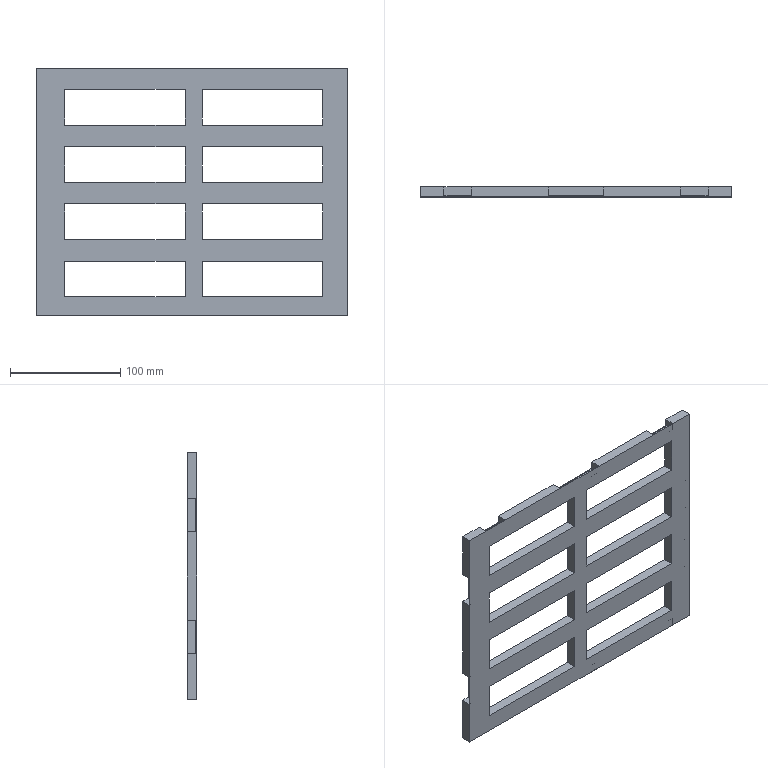Component | SolidWorks | 2011FeederTray-1 | 1 solid | 311 faces | box 282 x 9 x 224 mm | volume 294343 mm3 | plane 214 | spline 97
build123d program:
from build123d import *

# Parameters (mm, degrees)
SKETCH1_W            = 282
SKETCH1_H            = 224
BOSS_EXTRUDE1_DEPTH  = 9
SKETCH2_W            = 25
SKETCH2_H            = 7
SKETCH2_W_2          = 50
CUT_EXTRUDE1_DEPTH   = 8
SKETCH3_W            = 7
SKETCH3_H            = 30
CUT_EXTRUDE2_DEPTH   = 8
SKETCH4_W            = 7
SKETCH4_H            = 30
CUT_EXTRUDE3_DEPTH   = 8
SKETCH5_W            = 109.5
SKETCH5_H            = 32.5
CUT_EXTRUDE4_DEPTH   = 9
LPATTERN1_COUNT      = 4
LPATTERN1_PITCH      = 52
LPATTERN1_COUNT_DIR2 = 2
LPATTERN1_PITCH_DIR2 = 125
CUT_EXTRUDE5_DEPTH   = 2


with BuildPart() as part:
    # Sketch1 → Boss-Extrude1 (new body)
    with BuildSketch(Plane.XY):
        with Locations((141, 112)):
            Rectangle(SKETCH1_W, SKETCH1_H)
    extrude(amount=BOSS_EXTRUDE1_DEPTH)

    # Sketch2 → Cut-Extrude1 (cut)
    with BuildSketch(Plane(origin=(0, 0, 0), x_dir=(-1, 0, 0), z_dir=(0, 0, -1))):
        with Locations((-248.5, 3.5)):
            Rectangle(SKETCH2_W, SKETCH2_H)
        with Locations((-141, 3.5)):
            Rectangle(SKETCH2_W_2, SKETCH2_H)
        with Locations((-33.5, 3.5)):
            Rectangle(SKETCH2_W, SKETCH2_H)
    cut_extrude1 = extrude(amount=-CUT_EXTRUDE1_DEPTH, mode=Mode.SUBTRACT)

    # Mirror1: Cut-Extrude1 across plane
    add(cut_extrude1.mirror(Plane.ZX.offset(112)), mode=Mode.SUBTRACT)

    # Sketch3 → Cut-Extrude2 (cut)
    with BuildSketch(Plane(origin=(0, 0, 0), x_dir=(-1, 0, 0), z_dir=(0, 0, -1))):
        with Locations((-278.5, 167)):
            Rectangle(SKETCH3_W, SKETCH3_H)
        with Locations((-278.5, 57)):
            Rectangle(SKETCH3_W, SKETCH3_H)
    extrude(amount=-CUT_EXTRUDE2_DEPTH, mode=Mode.SUBTRACT)

    # Sketch4 → Cut-Extrude3 (cut)
    with BuildSketch(Plane(origin=(0, 0, 0), x_dir=(-1, 0, 0), z_dir=(0, 0, -1))):
        with Locations((-3.5, 152)):
            Rectangle(SKETCH4_W, SKETCH4_H)
        with Locations((-3.5, 87)):
            Rectangle(SKETCH4_W, SKETCH4_H)
    extrude(amount=-CUT_EXTRUDE3_DEPTH, mode=Mode.SUBTRACT)

    # Sketch5 → Cut-Extrude4 (cut)
    with BuildSketch(Plane(origin=(0, 0, 0), x_dir=(-1, 0, 0), z_dir=(0, 0, -1))):
        with Locations((-77, 191)):
            Rectangle(SKETCH5_W, SKETCH5_H)
    cut_extrude4 = extrude(amount=-CUT_EXTRUDE4_DEPTH, mode=Mode.SUBTRACT)

    # LPattern1: Cut-Extrude4 4 × 2
    with Locations(*[(j * LPATTERN1_PITCH_DIR2, -i * LPATTERN1_PITCH, 0) for i in range(LPATTERN1_COUNT) for j in range(LPATTERN1_COUNT_DIR2) if (i, j) != (0, 0)]):
        add(cut_extrude4, mode=Mode.SUBTRACT)

    # Sketch7 → Cut-Extrude5 (cut)
    # profile 1 of 6: a face of its own
    with BuildSketch(Plane(origin=(0, 0, 0), x_dir=(-1, 0, 0), z_dir=(0, 0, -1))):
        with BuildLine():
            add(Edge.make_bspline(
                [(-22.181, 112.918), (-22.127, 113.019), (-22.02, 113.218), (-21.9, 113.472), (-21.811, 113.669), (-21.753, 113.809), (-21.7, 113.94), (-21.659, 114.046), (-21.63, 114.13), (-21.607, 114.198), (-21.584, 114.273), (-21.56, 114.353), (-21.534, 114.439), (-21.509, 114.531), (-21.482, 114.629), (-21.465, 114.696), (-21.456, 114.731)],
                knots=[0, 0, 0, 0, 2.447, 4.852, 6.014, 7.097, 8.109, 9.044, 9.513, 10.031, 10.584, 11.185, 11.824, 12.505, 13.234, 14, 14, 14, 14], degree=3))
            add(Edge.make_bspline(
                [(-21.456, 114.731), (-21.484, 114.723), (-21.536, 114.708), (-21.611, 114.687), (-21.678, 114.666), (-21.738, 114.649), (-21.789, 114.631), (-21.833, 114.617), (-21.869, 114.603), (-21.89, 114.594), (-21.899, 114.59)],
                knots=[0, 0, 0, 0, 1.478, 2.813, 4.018, 5.09, 6.022, 6.809, 7.471, 8, 8, 8, 8], degree=3))
            Line((-21.899, 114.59), (-22.02, 114.716))
            add(Edge.make_bspline(
                [(-22.02, 114.716), (-22.028, 114.724), (-22.039, 114.737), (-22.055, 114.755), (-22.051, 114.772), (-22.044, 114.778), (-22.04, 114.781)],
                knots=[0, 0, 0, 0, 1.714, 2.651, 3.248, 4, 4, 4, 4], degree=3))
            add(Edge.make_bspline(
                [(-22.04, 114.781), (-22.038, 114.783), (-22.028, 114.787), (-22.014, 114.783), (-21.996, 114.783), (-21.977, 114.786), (-21.951, 114.791), (-21.917, 114.796), (-21.875, 114.803), (-21.826, 114.813), (-21.769, 114.824), (-21.729, 114.832), (-21.708, 114.837)],
                knots=[0, 0, 0, 0, 0.2376, 0.8998, 1.231, 1.808, 2.592, 3.618, 4.873, 6.357, 8.066, 10, 10, 10, 10], degree=3))
            Line((-21.708, 114.837), (-21.4, 114.897))
            Line((-21.4, 114.897), (-21.396, 115.541))
            Line((-21.396, 115.541), (-21.396, 115.657))
            add(Edge.make_bspline(
                [(-21.396, 115.657), (-21.396, 115.673), (-21.396, 115.702), (-21.396, 115.738), (-21.396, 115.762), (-21.396, 115.774), (-21.396, 115.778)],
                knots=[0, 0, 0, 0, 1.63, 2.84, 3.63, 4, 4, 4, 4], degree=3))
            add(Edge.make_bspline(
                [(-21.396, 115.778), (-21.396, 115.785), (-21.396, 115.805), (-21.398, 115.838), (-21.399, 115.883), (-21.402, 115.953), (-21.406, 116.039), (-21.41, 116.122), (-21.42, 116.187), (-21.431, 116.247), (-21.45, 116.32), (-21.464, 116.373), (-21.471, 116.402)],
                knots=[0, 0, 0, 0, 0.3663, 0.9103, 1.608, 2.483, 4.245, 5.679, 6.431, 7.392, 8.584, 10, 10, 10, 10], degree=3))
            Line((-21.471, 116.402), (-21.436, 116.442))
            Line((-21.436, 116.442), (-21.169, 116.11))
            add(Edge.make_bspline(
                [(-21.169, 116.11), (-21.179, 116.086), (-21.197, 116.038), (-21.224, 115.966), (-21.243, 115.887), (-21.253, 115.795), (-21.258, 115.687), (-21.263, 115.565), (-21.264, 115.439), (-21.264, 115.355), (-21.265, 115.315)],
                knots=[0, 0, 0, 0, 0.7826, 1.518, 2.286, 3.193, 4.257, 5.505, 6.797, 8, 8, 8, 8], degree=3))
            Line((-21.265, 115.315), (-21.27, 114.932))
            Line((-21.27, 114.932), (-21.159, 114.963))
            add(Edge.make_bspline(
                [(-21.159, 114.963), (-21.131, 114.97), (-21.08, 114.984), (-21.012, 115.011), (-20.956, 115.038), (-20.926, 115.062), (-20.913, 115.073)],
                knots=[0, 0, 0, 0, 1.246, 2.33, 3.232, 4, 4, 4, 4], degree=3))
            Line((-20.913, 115.073), (-20.772, 114.917))
            add(Edge.make_bspline(
                [(-20.772, 114.917), (-20.766, 114.909), (-20.757, 114.895), (-20.748, 114.871), (-20.76, 114.848), (-20.777, 114.847), (-20.787, 114.847)],
                knots=[0, 0, 0, 0, 1.175, 2.143, 2.906, 4, 4, 4, 4], degree=3))
            Line((-20.787, 114.847), (-20.836, 114.842))
            add(Edge.make_bspline(
                [(-20.836, 114.842), (-20.84, 114.841), (-20.852, 114.839), (-20.876, 114.834), (-20.912, 114.828), (-20.962, 114.819), (-21.023, 114.808), (-21.097, 114.794), (-21.184, 114.778), (-21.246, 114.767), (-21.279, 114.761)],
                knots=[0, 0, 0, 0, 0.2027, 0.6341, 1.294, 2.183, 3.301, 4.634, 6.209, 8, 8, 8, 8], degree=3))
            Line((-21.279, 114.761), (-21.279, 114.429))
            add(Edge.make_bspline(
                [(-21.279, 114.429), (-21.252, 114.41), (-21.199, 114.374), (-21.122, 114.323), (-21.05, 114.276), (-21.005, 114.247), (-20.983, 114.232)],
                knots=[0, 0, 0, 0, 1.123, 2.158, 3.121, 4, 4, 4, 4], degree=3))
            Line((-20.983, 114.232), (-20.922, 114.192))
            add(Edge.make_bspline(
                [(-20.922, 114.192), (-20.913, 114.184), (-20.897, 114.169), (-20.883, 114.138), (-20.878, 114.1), (-20.877, 114.073), (-20.877, 114.056)],
                knots=[0, 0, 0, 0, 0.9636, 1.761, 2.697, 4, 4, 4, 4], degree=3))
            Line((-20.877, 114.056), (-20.867, 113.845))
            add(Edge.make_bspline(
                [(-20.867, 113.845), (-20.867, 113.843), (-20.867, 113.837), (-20.867, 113.826), (-20.867, 113.808), (-20.868, 113.789), (-20.865, 113.77), (-20.879, 113.759), (-20.894, 113.776), (-20.902, 113.787), (-20.907, 113.795)],
                knots=[0, 0, 0, 0, 0.3193, 1.003, 2.098, 3.512, 4.706, 5.263, 6.212, 8, 8, 8, 8], degree=3))
            Line((-20.907, 113.795), (-20.942, 113.845))
            add(Edge.make_bspline(
                [(-20.942, 113.845), (-20.945, 113.849), (-20.955, 113.861), (-20.972, 113.887), (-20.998, 113.927), (-21.031, 113.981), (-21.075, 114.046), (-21.134, 114.122), (-21.206, 114.207), (-21.261, 114.266), (-21.29, 114.298)],
                knots=[0, 0, 0, 0, 0.2084, 0.6507, 1.307, 2.192, 3.302, 4.632, 6.2, 8, 8, 8, 8], degree=3))
            Line((-21.29, 114.298), (-21.325, 111.922))
            add(Edge.make_bspline(
                [(-21.325, 111.922), (-21.307, 111.961), (-21.272, 112.035), (-21.221, 112.144), (-21.175, 112.246), (-21.133, 112.34), (-21.095, 112.427), (-21.061, 112.508), (-21.032, 112.581), (-20.997, 112.671), (-20.957, 112.786), (-20.909, 112.935), (-20.862, 113.1), (-20.822, 113.246), (-20.791, 113.365), (-20.769, 113.451), (-20.75, 113.531), (-20.732, 113.605), (-20.716, 113.673), (-20.703, 113.735), (-20.69, 113.79), (-20.672, 113.89), (-20.646, 114.038), (-20.612, 114.238), (-20.582, 114.439), (-20.556, 114.606), (-20.538, 114.741), (-20.526, 114.851), (-20.516, 114.968), (-20.509, 115.07), (-20.503, 115.151), (-20.5, 115.207), (-20.496, 115.257), (-20.493, 115.301), (-20.491, 115.339), (-20.488, 115.372), (-20.486, 115.398), (-20.485, 115.414), (-20.484, 115.421)],
                knots=[0, 0, 0, 0, 1.269, 2.463, 3.577, 4.598, 5.544, 6.411, 7.192, 7.891, 9.29, 10.839, 12.544, 14.402, 15.344, 16.223, 17.039, 17.793, 18.485, 19.115, 19.683, 20.188, 22.137, 24.173, 26.219, 28.189, 29.206, 30.294, 31.469, 32.717, 33.334, 33.891, 34.388, 34.834, 35.212, 35.532, 35.799, 36, 36, 36, 36], degree=3))
            Line((-20.484, 115.421), (-20.479, 115.567))
            add(Edge.make_bspline(
                [(-20.479, 115.567), (-20.504, 115.561), (-20.551, 115.55), (-20.618, 115.533), (-20.679, 115.519), (-20.734, 115.504), (-20.783, 115.491), (-20.825, 115.479), (-20.861, 115.467), (-20.882, 115.459), (-20.892, 115.456)],
                knots=[0, 0, 0, 0, 1.417, 2.708, 3.884, 4.939, 5.892, 6.704, 7.409, 8, 8, 8, 8], degree=3))
            Line((-20.892, 115.456), (-21.003, 115.592))
            add(Edge.make_bspline(
                [(-21.003, 115.592), (-21.009, 115.599), (-21.021, 115.611), (-21.032, 115.629), (-21.032, 115.645), (-21.029, 115.653), (-21.028, 115.657)],
                knots=[0, 0, 0, 0, 1.585, 2.621, 3.38, 4, 4, 4, 4], degree=3))
            add(Edge.make_bspline(
                [(-21.028, 115.657), (-21.025, 115.659), (-21.014, 115.666), (-20.985, 115.666), (-20.94, 115.673), (-20.889, 115.674), (-20.835, 115.679), (-20.779, 115.686), (-20.711, 115.695), (-20.63, 115.709), (-20.536, 115.726), (-20.429, 115.745), (-20.31, 115.768), (-20.226, 115.785), (-20.182, 115.793)],
                knots=[0, 0, 0, 0, 0.1449, 0.5358, 1.175, 2.073, 2.681, 3.458, 4.427, 5.579, 6.903, 8.419, 10.118, 12, 12, 12, 12], degree=3))
            Line((-20.182, 115.793), (-19.8, 115.869))
            Line((-19.8, 115.869), (-19.734, 116.035))
            add(Edge.make_bspline(
                [(-19.734, 116.035), (-19.731, 116.045), (-19.725, 116.061), (-19.707, 116.082), (-19.682, 116.068), (-19.671, 116.054), (-19.664, 116.045)],
                knots=[0, 0, 0, 0, 1.266, 1.941, 2.633, 4, 4, 4, 4], degree=3))
            Line((-19.664, 116.045), (-19.538, 115.864))
            add(Edge.make_bspline(
                [(-19.538, 115.864), (-19.532, 115.854), (-19.523, 115.838), (-19.519, 115.82), (-19.518, 115.814)],
                knots=[0, 0, 0, 0, 1.232, 2, 2, 2, 2], degree=3))
            add(Edge.make_bspline(
                [(-19.518, 115.814), (-19.518, 115.81), (-19.519, 115.804), (-19.523, 115.796), (-19.53, 115.788), (-19.541, 115.779), (-19.556, 115.765), (-19.586, 115.744), (-19.623, 115.704), (-19.649, 115.65), (-19.668, 115.595), (-19.686, 115.538), (-19.707, 115.467), (-19.721, 115.414), (-19.729, 115.385)],
                knots=[0, 0, 0, 0, 0.2403, 0.4611, 0.6553, 0.9922, 1.498, 2.174, 3.699, 5.432, 6.536, 7.992, 9.819, 12, 12, 12, 12], degree=3))
            Line((-19.729, 115.385), (-19.915, 114.646))
            Line((-19.915, 114.646), (-19.659, 114.706))
            Line((-19.659, 114.706), (-19.598, 114.842))
            add(Edge.make_bspline(
                [(-19.598, 114.842), (-19.595, 114.849), (-19.588, 114.862), (-19.567, 114.871), (-19.545, 114.858), (-19.534, 114.845), (-19.528, 114.837)],
                knots=[0, 0, 0, 0, 1.047, 1.789, 2.654, 4, 4, 4, 4], degree=3))
            Line((-19.528, 114.837), (-19.417, 114.675))
            add(Edge.make_bspline(
                [(-19.417, 114.675), (-19.413, 114.667), (-19.406, 114.653), (-19.398, 114.635), (-19.393, 114.623), (-19.39, 114.614), (-19.388, 114.606), (-19.391, 114.602), (-19.392, 114.6)],
                knots=[0, 0, 0, 0, 2.075, 3.445, 4.327, 5.017, 5.512, 6, 6, 6, 6], degree=3))
            add(Edge.make_bspline(
                [(-19.392, 114.6), (-19.394, 114.597), (-19.398, 114.589), (-19.412, 114.579), (-19.429, 114.564), (-19.462, 114.544), (-19.501, 114.513), (-19.535, 114.459), (-19.556, 114.39), (-19.573, 114.33), (-19.587, 114.28), (-19.595, 114.245), (-19.606, 114.204), (-19.617, 114.156), (-19.632, 114.101), (-19.649, 114.039), (-19.665, 113.971), (-19.685, 113.895), (-19.707, 113.813), (-19.732, 113.725), (-19.763, 113.631), (-19.796, 113.53), (-19.835, 113.423), (-19.875, 113.308), (-19.922, 113.189), (-19.954, 113.107), (-19.971, 113.065)],
                knots=[0, 0, 0, 0, 0.1551, 0.3909, 0.72, 1.146, 2.032, 2.864, 3.847, 5.154, 5.566, 6.087, 6.698, 7.417, 8.228, 9.152, 10.171, 11.292, 12.518, 13.839, 15.274, 16.804, 18.446, 20.194, 22.049, 24, 24, 24, 24], degree=3))
            add(Edge.make_bspline(
                [(-19.971, 113.065), (-19.946, 113.007), (-19.898, 112.898), (-19.824, 112.745), (-19.755, 112.607), (-19.69, 112.484), (-19.625, 112.378), (-19.556, 112.29), (-19.486, 112.217), (-19.408, 112.16), (-19.321, 112.117), (-19.221, 112.08), (-19.106, 112.047), (-19.023, 112.031), (-18.979, 112.023)],
                knots=[0, 0, 0, 0, 1.467, 2.802, 4.014, 5.098, 6.071, 6.942, 7.732, 8.449, 9.184, 10.016, 10.953, 12, 12, 12, 12], degree=3))
            Line((-18.979, 112.023), (-18.984, 111.922))
            Line((-18.984, 111.922), (-19.613, 111.897))
            add(Edge.make_bspline(
                [(-19.613, 111.897), (-19.624, 111.922), (-19.648, 111.977), (-19.686, 112.067), (-19.731, 112.172), (-19.782, 112.291), (-19.841, 112.424), (-19.905, 112.573), (-19.976, 112.736), (-20.025, 112.85), (-20.051, 112.909)],
                knots=[0, 0, 0, 0, 0.594, 1.307, 2.131, 3.074, 4.13, 5.303, 6.595, 8, 8, 8, 8], degree=3))
            add(Edge.make_bspline(
                [(-20.051, 112.909), (-20.097, 112.826), (-20.188, 112.661), (-20.308, 112.458), (-20.412, 112.298), (-20.503, 112.178), (-20.606, 112.057), (-20.717, 111.937), (-20.831, 111.824), (-20.94, 111.723), (-21.042, 111.637), (-21.111, 111.588), (-21.144, 111.565)],
                knots=[0, 0, 0, 0, 1.626, 3.227, 4.039, 4.898, 5.806, 6.765, 7.703, 8.55, 9.319, 10, 10, 10, 10], degree=3))
            Line((-21.144, 111.565), (-21.179, 111.645))
            add(Edge.make_bspline(
                [(-21.179, 111.645), (-21.156, 111.666), (-21.107, 111.709), (-21.03, 111.783), (-20.943, 111.869), (-20.846, 111.965), (-20.745, 112.074), (-20.645, 112.197), (-20.548, 112.335), (-20.453, 112.483), (-20.363, 112.638), (-20.276, 112.791), (-20.196, 112.943), (-20.146, 113.045), (-20.122, 113.095)],
                knots=[0, 0, 0, 0, 0.606, 1.309, 2.121, 3.031, 4.025, 5.077, 6.194, 7.376, 8.582, 9.752, 10.892, 12, 12, 12, 12], degree=3))
            add(Edge.make_bspline(
                [(-20.122, 113.095), (-20.141, 113.141), (-20.176, 113.228), (-20.226, 113.352), (-20.271, 113.461), (-20.309, 113.557), (-20.341, 113.639), (-20.367, 113.707), (-20.388, 113.76), (-20.415, 113.836), (-20.452, 113.94), (-20.487, 114.03), (-20.505, 114.077)],
                knots=[0, 0, 0, 0, 1.413, 2.674, 3.798, 4.78, 5.609, 6.299, 6.846, 7.245, 8.591, 10, 10, 10, 10], degree=3))
            add(Edge.make_bspline(
                [(-20.505, 114.077), (-20.513, 114.039), (-20.528, 113.968), (-20.549, 113.867), (-20.569, 113.779), (-20.585, 113.702), (-20.599, 113.637), (-20.611, 113.584), (-20.621, 113.543), (-20.628, 113.51), (-20.636, 113.48), (-20.646, 113.445), (-20.656, 113.402), (-20.671, 113.351), (-20.689, 113.293), (-20.706, 113.226), (-20.728, 113.152), (-20.76, 113.043), (-20.802, 112.905), (-20.857, 112.742), (-20.916, 112.586), (-20.977, 112.435), (-21.044, 112.285), (-21.119, 112.135), (-21.2, 111.981), (-21.26, 111.879), (-21.29, 111.827)],
                knots=[0, 0, 0, 0, 1.153, 2.185, 3.095, 3.875, 4.547, 5.091, 5.513, 5.812, 6.09, 6.454, 6.902, 7.429, 8.037, 8.735, 9.513, 10.369, 12.143, 13.854, 15.53, 17.145, 18.767, 20.441, 22.193, 24, 24, 24, 24], degree=3))
            Line((-21.29, 111.827), (-21.33, 111.867))
            Line((-21.33, 111.867), (-21.34, 111.706))
            add(Edge.make_bspline(
                [(-21.34, 111.706), (-21.342, 111.69), (-21.346, 111.661), (-21.358, 111.629), (-21.37, 111.611), (-21.381, 111.604), (-21.393, 111.613), (-21.398, 111.62), (-21.4, 111.625)],
                knots=[0, 0, 0, 0, 2.023, 3.752, 4.395, 4.813, 5.287, 6, 6, 6, 6], degree=3))
            add(Edge.make_bspline(
                [(-21.4, 111.625), (-21.405, 111.63), (-21.416, 111.643), (-21.419, 111.66), (-21.42, 111.67)],
                knots=[0, 0, 0, 0, 0.8287, 2, 2, 2, 2], degree=3))
            Line((-21.42, 111.67), (-21.451, 111.761))
            Line((-21.451, 111.761), (-21.491, 111.876))
            add(Edge.make_bspline(
                [(-21.491, 111.876), (-21.498, 111.897), (-21.51, 111.932), (-21.524, 111.977), (-21.533, 112.007), (-21.536, 112.023), (-21.537, 112.028)],
                knots=[0, 0, 0, 0, 1.61, 2.815, 3.597, 4, 4, 4, 4], degree=3))
            add(Edge.make_bspline(
                [(-21.537, 112.028), (-21.536, 112.031), (-21.534, 112.04), (-21.529, 112.056), (-21.519, 112.076), (-21.506, 112.102), (-21.492, 112.133), (-21.479, 112.171), (-21.469, 112.214), (-21.458, 112.283), (-21.446, 112.382), (-21.442, 112.466), (-21.441, 112.511)],
                knots=[0, 0, 0, 0, 0.2147, 0.5323, 0.9951, 1.578, 2.283, 3.075, 3.969, 4.958, 7.267, 10, 10, 10, 10], degree=3))
            Line((-21.441, 112.511), (-21.406, 114.408))
            add(Edge.make_bspline(
                [(-21.406, 114.408), (-21.425, 114.349), (-21.462, 114.237), (-21.518, 114.079), (-21.571, 113.939), (-21.64, 113.774), (-21.733, 113.575), (-21.853, 113.334), (-21.986, 113.092), (-22.09, 112.939), (-22.141, 112.863)],
                knots=[0, 0, 0, 0, 0.8678, 1.649, 2.348, 2.962, 4.143, 5.422, 6.725, 8, 8, 8, 8], degree=3))
            Line((-22.141, 112.863), (-22.181, 112.918))
        make_face()
        with BuildLine():
            Line((-20.474, 114.273), (-20.404, 114.258))
            add(Edge.make_bspline(
                [(-20.404, 114.258), (-20.401, 114.23), (-20.396, 114.173), (-20.388, 114.11), (-20.377, 114.071), (-20.372, 114.051), (-20.364, 114.028), (-20.353, 113.999), (-20.341, 113.965), (-20.326, 113.925), (-20.309, 113.881), (-20.289, 113.832), (-20.268, 113.777), (-20.244, 113.718), (-20.217, 113.654), (-20.189, 113.584), (-20.157, 113.509), (-20.125, 113.429), (-20.088, 113.345), (-20.064, 113.286), (-20.051, 113.256)],
                knots=[0, 0, 0, 0, 1.404, 2.92, 3.167, 3.494, 3.92, 4.441, 5.058, 5.759, 6.568, 7.461, 8.449, 9.522, 10.706, 11.97, 13.347, 14.803, 16.348, 18, 18, 18, 18], degree=3))
            add(Edge.make_bspline(
                [(-20.051, 113.256), (-20.037, 113.294), (-20.011, 113.367), (-19.973, 113.474), (-19.94, 113.572), (-19.909, 113.661), (-19.883, 113.743), (-19.859, 113.817), (-19.84, 113.883), (-19.817, 113.963), (-19.791, 114.068), (-19.756, 114.208), (-19.718, 114.369), (-19.693, 114.484), (-19.679, 114.545)],
                knots=[0, 0, 0, 0, 1.084, 2.087, 3.016, 3.862, 4.633, 5.324, 5.936, 6.47, 7.557, 8.841, 10.327, 12, 12, 12, 12], degree=3))
            Line((-19.679, 114.545), (-19.926, 114.499))
            Line((-19.926, 114.499), (-19.996, 114.373))
            add(Edge.make_bspline(
                [(-19.996, 114.373), (-20.002, 114.366), (-20.01, 114.354), (-20.02, 114.333), (-20.031, 114.339), (-20.039, 114.348), (-20.053, 114.363), (-20.062, 114.376), (-20.067, 114.384)],
                knots=[0, 0, 0, 0, 1.694, 2.508, 2.81, 3.483, 4.524, 6, 6, 6, 6], degree=3))
            Line((-20.067, 114.384), (-20.137, 114.474))
            add(Edge.make_bspline(
                [(-20.137, 114.474), (-20.144, 114.482), (-20.155, 114.495), (-20.169, 114.513), (-20.177, 114.528), (-20.177, 114.536), (-20.177, 114.54)],
                knots=[0, 0, 0, 0, 1.537, 2.706, 3.505, 4, 4, 4, 4], degree=3))
            add(Edge.make_bspline(
                [(-20.177, 114.54), (-20.176, 114.542), (-20.174, 114.548), (-20.165, 114.559), (-20.152, 114.573), (-20.126, 114.597), (-20.092, 114.634), (-20.065, 114.68), (-20.045, 114.722), (-20.031, 114.761), (-20.017, 114.805), (-19.998, 114.874), (-19.974, 114.966), (-19.949, 115.059), (-19.928, 115.13), (-19.916, 115.178), (-19.904, 115.218), (-19.898, 115.243), (-19.895, 115.254)],
                knots=[0, 0, 0, 0, 0.1507, 0.4139, 0.8256, 1.356, 2.591, 3.882, 4.608, 5.46, 6.423, 7.503, 9.845, 12.258, 13.42, 14.434, 15.291, 16, 16, 16, 16], degree=3))
            Line((-19.895, 115.254), (-19.8, 115.697))
            Line((-19.8, 115.697), (-20.313, 115.592))
            add(Edge.make_bspline(
                [(-20.313, 115.592), (-20.316, 115.566), (-20.322, 115.51), (-20.33, 115.418), (-20.341, 115.312), (-20.351, 115.196), (-20.362, 115.08), (-20.372, 114.972), (-20.385, 114.878), (-20.394, 114.805), (-20.403, 114.748), (-20.41, 114.7), (-20.419, 114.645), (-20.427, 114.584), (-20.438, 114.516), (-20.449, 114.441), (-20.461, 114.359), (-20.47, 114.302), (-20.474, 114.273)],
                knots=[0, 0, 0, 0, 0.9386, 2.048, 3.328, 4.779, 6.239, 7.539, 8.696, 9.693, 10.192, 10.773, 11.436, 12.188, 13.015, 13.931, 14.92, 16, 16, 16, 16], degree=3))
        make_face(mode=Mode.SUBTRACT)
    # profile 2 of 6: a face of its own
    with BuildSketch(Plane(origin=(0, 0, 0), x_dir=(-1, 0, 0), z_dir=(0, 0, -1))):
        with BuildLine():
            Line((-17.612, 113.18), (-17.607, 115.552))
            add(Edge.make_bspline(
                [(-17.607, 115.552), (-17.653, 115.544), (-17.739, 115.529), (-17.858, 115.506), (-17.96, 115.484), (-18.022, 115.468), (-18.05, 115.461)],
                knots=[0, 0, 0, 0, 1.233, 2.307, 3.232, 4, 4, 4, 4], degree=3))
            Line((-18.05, 115.461), (-18.191, 115.587))
            add(Edge.make_bspline(
                [(-18.191, 115.587), (-18.198, 115.592), (-18.209, 115.602), (-18.224, 115.615), (-18.233, 115.626), (-18.238, 115.639), (-18.233, 115.654), (-18.225, 115.663), (-18.221, 115.667)],
                knots=[0, 0, 0, 0, 1.48, 2.617, 3.426, 3.975, 4.914, 6, 6, 6, 6], degree=3))
            add(Edge.make_bspline(
                [(-18.221, 115.667), (-18.218, 115.668), (-18.208, 115.672), (-18.186, 115.675), (-18.153, 115.678), (-18.126, 115.681), (-18.111, 115.682)],
                knots=[0, 0, 0, 0, 0.3381, 1.125, 2.335, 4, 4, 4, 4], degree=3))
            Line((-18.111, 115.682), (-18.025, 115.682))
            add(Edge.make_bspline(
                [(-18.025, 115.682), (-18.013, 115.683), (-17.982, 115.684), (-17.925, 115.69), (-17.848, 115.699), (-17.749, 115.71), (-17.63, 115.727), (-17.49, 115.745), (-17.329, 115.767), (-17.153, 115.793), (-16.976, 115.818), (-16.812, 115.843), (-16.665, 115.865), (-16.537, 115.886), (-16.428, 115.905), (-16.337, 115.921), (-16.265, 115.935), (-16.195, 115.951), (-16.124, 115.971), (-16.051, 115.997), (-15.989, 116.023), (-15.953, 116.045), (-15.936, 116.055)],
                knots=[0, 0, 0, 0, 0.3364, 0.8707, 1.604, 2.535, 3.664, 4.992, 6.519, 8.245, 9.985, 11.55, 12.938, 14.158, 15.195, 16.063, 16.755, 17.273, 18.095, 18.815, 19.451, 20, 20, 20, 20], degree=3))
            Line((-15.936, 116.055), (-15.795, 115.899))
            add(Edge.make_bspline(
                [(-15.795, 115.899), (-15.786, 115.886), (-15.771, 115.865), (-15.755, 115.835), (-15.766, 115.81), (-15.781, 115.809), (-15.79, 115.808)],
                knots=[0, 0, 0, 0, 1.601, 2.596, 3.2, 4, 4, 4, 4], degree=3))
            Line((-15.79, 115.808), (-16.389, 115.737))
            Line((-16.389, 115.737), (-16.389, 113.407))
            add(Edge.make_bspline(
                [(-16.389, 113.407), (-16.341, 113.417), (-16.251, 113.437), (-16.124, 113.467), (-16.01, 113.495), (-15.91, 113.524), (-15.823, 113.55), (-15.751, 113.576), (-15.692, 113.601), (-15.658, 113.62), (-15.644, 113.628)],
                knots=[0, 0, 0, 0, 1.489, 2.833, 4.041, 5.107, 6.029, 6.818, 7.476, 8, 8, 8, 8], degree=3))
            Line((-15.644, 113.628), (-15.477, 113.452))
            add(Edge.make_bspline(
                [(-15.477, 113.452), (-15.471, 113.444), (-15.46, 113.431), (-15.451, 113.412), (-15.454, 113.4), (-15.456, 113.392), (-15.464, 113.39), (-15.474, 113.387), (-15.49, 113.384), (-15.511, 113.381), (-15.539, 113.375), (-15.572, 113.37), (-15.611, 113.363), (-15.639, 113.359), (-15.654, 113.357)],
                knots=[0, 0, 0, 0, 1.437, 2.25, 2.723, 3.067, 3.247, 3.733, 4.447, 5.431, 6.689, 8.177, 9.973, 12, 12, 12, 12], degree=3))
            Line((-15.654, 113.357), (-16.389, 113.236))
            Line((-16.389, 113.236), (-16.389, 112.053))
            Line((-16.389, 112.053), (-16.394, 111.695))
            add(Edge.make_bspline(
                [(-16.394, 111.695), (-16.394, 111.675), (-16.394, 111.64), (-16.399, 111.598), (-16.402, 111.569), (-16.421, 111.559), (-16.435, 111.573), (-16.447, 111.592), (-16.461, 111.623), (-16.47, 111.647), (-16.474, 111.66)],
                knots=[0, 0, 0, 0, 1.902, 3.231, 4.038, 4.422, 4.904, 5.638, 6.665, 8, 8, 8, 8], degree=3))
            Line((-16.474, 111.66), (-16.56, 111.887))
            add(Edge.make_bspline(
                [(-16.56, 111.887), (-16.566, 111.902), (-16.577, 111.928), (-16.59, 111.962), (-16.597, 111.986), (-16.604, 112.002), (-16.602, 112.018), (-16.596, 112.038), (-16.587, 112.068), (-16.579, 112.09), (-16.575, 112.103)],
                knots=[0, 0, 0, 0, 1.692, 2.975, 3.861, 4.325, 4.744, 5.5, 6.568, 8, 8, 8, 8], degree=3))
            add(Edge.make_bspline(
                [(-16.575, 112.103), (-16.572, 112.115), (-16.567, 112.14), (-16.56, 112.181), (-16.551, 112.23), (-16.547, 112.266), (-16.544, 112.284)],
                knots=[0, 0, 0, 0, 0.7638, 1.671, 2.756, 4, 4, 4, 4], degree=3))
            Line((-16.544, 112.284), (-16.535, 112.365))
            add(Edge.make_bspline(
                [(-16.535, 112.365), (-16.533, 112.382), (-16.531, 112.412), (-16.526, 112.454), (-16.525, 112.486), (-16.525, 112.504), (-16.524, 112.511)],
                knots=[0, 0, 0, 0, 1.389, 2.513, 3.389, 4, 4, 4, 4], degree=3))
            Line((-16.524, 112.511), (-16.524, 113.22))
            add(Edge.make_bspline(
                [(-16.524, 113.22), (-16.583, 113.208), (-16.699, 113.184), (-16.867, 113.15), (-17.025, 113.117), (-17.175, 113.087), (-17.315, 113.057), (-17.446, 113.029), (-17.568, 113.005), (-17.68, 112.979), (-17.784, 112.957), (-17.878, 112.937), (-17.963, 112.917), (-18.038, 112.901), (-18.105, 112.885), (-18.162, 112.872), (-18.21, 112.86), (-18.239, 112.852), (-18.252, 112.848)],
                knots=[0, 0, 0, 0, 1.641, 3.192, 4.66, 6.039, 7.337, 8.552, 9.683, 10.72, 11.68, 12.55, 13.34, 14.039, 14.657, 15.191, 15.636, 16, 16, 16, 16], degree=3))
            Line((-18.252, 112.848), (-18.393, 112.984))
            add(Edge.make_bspline(
                [(-18.393, 112.984), (-18.401, 112.993), (-18.413, 113.007), (-18.43, 113.027), (-18.423, 113.043), (-18.417, 113.05), (-18.413, 113.055)],
                knots=[0, 0, 0, 0, 1.783, 2.606, 3.176, 4, 4, 4, 4], degree=3))
            Line((-18.413, 113.055), (-18.176, 113.09))
            Line((-18.176, 113.09), (-17.612, 113.18))
        make_face()
        with BuildLine():
            Line((-17.476, 113.905), (-17.476, 113.196))
            Line((-17.476, 113.196), (-16.524, 113.377))
            Line((-16.524, 113.377), (-16.524, 115.713))
            Line((-16.524, 115.713), (-17.476, 115.567))
            Line((-17.476, 115.567), (-17.476, 114.862))
            add(Edge.make_bspline(
                [(-17.476, 114.862), (-17.439, 114.871), (-17.369, 114.888), (-17.271, 114.914), (-17.186, 114.937), (-17.114, 114.958), (-17.054, 114.975), (-17.007, 114.992), (-16.972, 115.004), (-16.954, 115.014), (-16.947, 115.018)],
                knots=[0, 0, 0, 0, 1.649, 3.122, 4.398, 5.49, 6.392, 7.113, 7.647, 8, 8, 8, 8], degree=3))
            Line((-16.947, 115.018), (-16.867, 115.063))
            Line((-16.867, 115.063), (-16.721, 114.942))
            add(Edge.make_bspline(
                [(-16.721, 114.942), (-16.716, 114.937), (-16.706, 114.928), (-16.696, 114.913), (-16.69, 114.901), (-16.69, 114.887), (-16.701, 114.873), (-16.714, 114.869), (-16.721, 114.867)],
                knots=[0, 0, 0, 0, 1.326, 2.33, 3.132, 3.699, 4.728, 6, 6, 6, 6], degree=3))
            Line((-16.721, 114.867), (-17.476, 114.701))
            Line((-17.476, 114.701), (-17.476, 114.062))
            add(Edge.make_bspline(
                [(-17.476, 114.062), (-17.445, 114.071), (-17.385, 114.088), (-17.302, 114.113), (-17.229, 114.134), (-17.167, 114.153), (-17.116, 114.169), (-17.074, 114.181), (-17.044, 114.192), (-17.005, 114.205), (-16.95, 114.233), (-16.903, 114.262), (-16.877, 114.278)],
                knots=[0, 0, 0, 0, 1.532, 2.893, 4.085, 5.096, 5.938, 6.609, 7.114, 7.435, 8.562, 10, 10, 10, 10], degree=3))
            Line((-16.877, 114.278), (-16.721, 114.172))
            add(Edge.make_bspline(
                [(-16.721, 114.172), (-16.711, 114.163), (-16.694, 114.148), (-16.683, 114.12), (-16.689, 114.094), (-16.703, 114.089), (-16.711, 114.086)],
                knots=[0, 0, 0, 0, 1.415, 2.441, 3.202, 4, 4, 4, 4], degree=3))
            Line((-16.711, 114.086), (-16.993, 114.026))
            Line((-16.993, 114.026), (-17.476, 113.905))
        make_face(mode=Mode.SUBTRACT)
    # profile 3 of 6: a face of its own
    with BuildSketch(Plane(origin=(0, 0, 0), x_dir=(-1, 0, 0), z_dir=(0, 0, -1))):
        with BuildLine():
            add(Edge.make_bspline(
                [(-14.855, 111.655), (-14.851, 111.659), (-14.84, 111.668), (-14.82, 111.687), (-14.791, 111.713), (-14.755, 111.747), (-14.712, 111.788), (-14.66, 111.836), (-14.601, 111.892), (-14.534, 111.953), (-14.464, 112.023), (-14.394, 112.101), (-14.324, 112.187), (-14.257, 112.281), (-14.19, 112.382), (-14.124, 112.491), (-14.059, 112.607), (-13.996, 112.73), (-13.936, 112.854), (-13.88, 112.976), (-13.828, 113.094), (-13.782, 113.209), (-13.741, 113.32), (-13.704, 113.427), (-13.673, 113.531), (-13.647, 113.631), (-13.624, 113.725), (-13.604, 113.812), (-13.586, 113.891), (-13.569, 113.963), (-13.556, 114.027), (-13.544, 114.083), (-13.534, 114.132), (-13.52, 114.213), (-13.502, 114.329), (-13.488, 114.455), (-13.48, 114.553), (-13.473, 114.62), (-13.469, 114.68), (-13.467, 114.718), (-13.466, 114.736)],
                knots=[0, 0, 0, 0, 0.1848, 0.4846, 0.9057, 1.448, 2.099, 2.866, 3.76, 4.763, 5.858, 6.995, 8.2, 9.467, 10.785, 12.178, 13.634, 15.158, 16.689, 18.158, 19.563, 20.916, 22.211, 23.45, 24.634, 25.762, 26.828, 27.798, 28.694, 29.496, 30.212, 30.845, 31.386, 31.849, 33.531, 35.212, 36.022, 36.75, 37.412, 38, 38, 38, 38], degree=3))
            add(Edge.make_bspline(
                [(-13.466, 114.736), (-13.466, 114.759), (-13.467, 114.806), (-13.473, 114.852), (-13.476, 114.877)],
                knots=[0, 0, 0, 0, 0.9601, 2, 2, 2, 2], degree=3))
            add(Edge.make_bspline(
                [(-13.476, 114.877), (-13.571, 114.868), (-13.759, 114.85), (-14.038, 114.81), (-14.315, 114.764), (-14.497, 114.725), (-14.588, 114.706)],
                knots=[0, 0, 0, 0, 1.01, 2.013, 3.007, 4, 4, 4, 4], degree=3))
            Line((-14.588, 114.706), (-14.785, 114.892))
            add(Edge.make_bspline(
                [(-14.785, 114.892), (-14.791, 114.896), (-14.8, 114.903), (-14.808, 114.916), (-14.809, 114.928), (-14.807, 114.934), (-14.805, 114.937)],
                knots=[0, 0, 0, 0, 1.542, 2.495, 3.259, 4, 4, 4, 4], degree=3))
            add(Edge.make_bspline(
                [(-14.805, 114.937), (-14.804, 114.938), (-14.8, 114.942), (-14.787, 114.943), (-14.768, 114.947), (-14.739, 114.95), (-14.7, 114.954), (-14.649, 114.957), (-14.584, 114.96), (-14.519, 114.962), (-14.453, 114.966), (-14.383, 114.971), (-14.293, 114.979), (-14.185, 114.991), (-14.058, 115.005), (-13.913, 115.022), (-13.749, 115.041), (-13.633, 115.056), (-13.572, 115.063)],
                knots=[0, 0, 0, 0, 0.06155, 0.2201, 0.473, 0.8319, 1.324, 1.989, 2.826, 3.826, 4.491, 5.397, 6.555, 7.957, 9.601, 11.488, 13.618, 16, 16, 16, 16], degree=3))
            Line((-13.572, 115.063), (-13.028, 115.129))
            add(Edge.make_bspline(
                [(-13.028, 115.129), (-12.97, 115.136), (-12.858, 115.149), (-12.698, 115.173), (-12.553, 115.197), (-12.423, 115.224), (-12.308, 115.251), (-12.209, 115.28), (-12.124, 115.31), (-12.074, 115.334), (-12.051, 115.345)],
                knots=[0, 0, 0, 0, 1.406, 2.691, 3.859, 4.914, 5.855, 6.678, 7.392, 8, 8, 8, 8], degree=3))
            Line((-12.051, 115.345), (-11.86, 115.133))
            add(Edge.make_bspline(
                [(-11.86, 115.133), (-11.855, 115.124), (-11.844, 115.108), (-11.843, 115.082), (-11.854, 115.061), (-11.868, 115.059), (-11.875, 115.058)],
                knots=[0, 0, 0, 0, 1.315, 2.337, 3.128, 4, 4, 4, 4], degree=3))
            Line((-11.875, 115.058), (-11.956, 115.053))
            add(Edge.make_bspline(
                [(-11.956, 115.053), (-11.998, 115.05), (-12.088, 115.043), (-12.227, 115.03), (-12.379, 115.016), (-12.542, 114.997), (-12.717, 114.977), (-12.905, 114.955), (-13.103, 114.929), (-13.24, 114.911), (-13.31, 114.902)],
                knots=[0, 0, 0, 0, 0.7551, 1.577, 2.47, 3.435, 4.47, 5.577, 6.755, 8, 8, 8, 8], degree=3))
            Line((-13.31, 114.902), (-13.199, 114.696))
            add(Edge.make_bspline(
                [(-13.199, 114.696), (-13.208, 114.681), (-13.226, 114.652), (-13.249, 114.609), (-13.268, 114.571), (-13.288, 114.523), (-13.305, 114.455), (-13.314, 114.399), (-13.32, 114.368)],
                knots=[0, 0, 0, 0, 0.9061, 1.73, 2.451, 3.095, 4.411, 6, 6, 6, 6], degree=3))
            Line((-13.32, 114.368), (-13.355, 114.177))
            Line((-13.355, 114.177), (-13.38, 114.046))
            add(Edge.make_bspline(
                [(-13.38, 114.046), (-13.326, 114.052), (-13.211, 114.066), (-13.097, 114.09), (-13.038, 114.102)],
                knots=[0, 0, 0, 0, 0.9496, 2, 2, 2, 2], degree=3))
            Line((-13.038, 114.102), (-12.887, 114.137))
            Line((-12.887, 114.137), (-12.741, 114.167))
            Line((-12.741, 114.167), (-12.64, 114.368))
            add(Edge.make_bspline(
                [(-12.64, 114.368), (-12.636, 114.377), (-12.629, 114.391), (-12.605, 114.399), (-12.582, 114.384), (-12.571, 114.368), (-12.565, 114.358)],
                knots=[0, 0, 0, 0, 1.059, 1.783, 2.663, 4, 4, 4, 4], degree=3))
            Line((-12.565, 114.358), (-12.439, 114.162))
            add(Edge.make_bspline(
                [(-12.439, 114.162), (-12.437, 114.157), (-12.433, 114.146), (-12.429, 114.129), (-12.425, 114.114), (-12.421, 114.102), (-12.423, 114.088), (-12.429, 114.081), (-12.434, 114.077)],
                knots=[0, 0, 0, 0, 1.125, 2.283, 3.348, 4.151, 4.889, 6, 6, 6, 6], degree=3))
            add(Edge.make_bspline(
                [(-12.434, 114.077), (-12.439, 114.071), (-12.455, 114.056), (-12.485, 114.03), (-12.518, 113.991), (-12.544, 113.94), (-12.563, 113.884), (-12.575, 113.84), (-12.582, 113.806), (-12.586, 113.779), (-12.592, 113.744), (-12.6, 113.702), (-12.608, 113.651), (-12.617, 113.592), (-12.627, 113.525), (-12.638, 113.45), (-12.651, 113.368), (-12.666, 113.281), (-12.683, 113.188), (-12.702, 113.09), (-12.722, 112.986), (-12.746, 112.877), (-12.77, 112.762), (-12.797, 112.644), (-12.824, 112.528), (-12.85, 112.417), (-12.877, 112.314), (-12.904, 112.219), (-12.93, 112.132), (-12.956, 112.053), (-12.981, 111.982), (-13.007, 111.919), (-13.031, 111.864), (-13.053, 111.816), (-13.071, 111.775), (-13.087, 111.742), (-13.101, 111.717), (-13.113, 111.699), (-13.12, 111.687), (-13.133, 111.679), (-13.152, 111.697), (-13.159, 111.712), (-13.164, 111.721)],
                knots=[0, 0, 0, 0, 0.3687, 1.033, 1.847, 2.738, 3.662, 4.583, 4.879, 5.29, 5.843, 6.513, 7.311, 8.237, 9.292, 10.475, 11.764, 13.139, 14.612, 16.157, 17.811, 19.54, 21.364, 23.276, 25.167, 26.943, 28.595, 30.124, 31.528, 32.821, 33.99, 35.05, 35.984, 36.798, 37.498, 38.068, 38.519, 38.847, 39.07, 39.173, 39.511, 40, 40, 40, 40], degree=3))
            Line((-13.164, 111.721), (-13.184, 111.771))
            add(Edge.make_bspline(
                [(-13.184, 111.771), (-13.198, 111.803), (-13.224, 111.865), (-13.263, 111.953), (-13.299, 112.034), (-13.335, 112.108), (-13.373, 112.184), (-13.42, 112.264), (-13.474, 112.353), (-13.515, 112.413), (-13.537, 112.446)],
                knots=[0, 0, 0, 0, 1.107, 2.115, 3.042, 3.874, 4.723, 5.697, 6.782, 8, 8, 8, 8], degree=3))
            Line((-13.537, 112.446), (-13.496, 112.511))
            Line((-13.496, 112.511), (-13.27, 112.284))
            add(Edge.make_bspline(
                [(-13.27, 112.284), (-13.253, 112.267), (-13.223, 112.237), (-13.185, 112.197), (-13.16, 112.176), (-13.146, 112.158), (-13.129, 112.165), (-13.122, 112.173), (-13.118, 112.179)],
                knots=[0, 0, 0, 0, 2.122, 3.668, 4.653, 5.065, 5.424, 6, 6, 6, 6], degree=3))
            add(Edge.make_bspline(
                [(-13.118, 112.179), (-13.115, 112.186), (-13.105, 112.207), (-13.087, 112.25), (-13.064, 112.312), (-13.033, 112.393), (-13, 112.491), (-12.967, 112.604), (-12.936, 112.731), (-12.907, 112.869), (-12.878, 113.008), (-12.854, 113.142), (-12.83, 113.265), (-12.81, 113.377), (-12.793, 113.475), (-12.779, 113.556), (-12.769, 113.618), (-12.763, 113.654), (-12.761, 113.669)],
                knots=[0, 0, 0, 0, 0.2571, 0.7374, 1.428, 2.34, 3.43, 4.659, 6.019, 7.529, 9.05, 10.465, 11.769, 12.968, 14.016, 14.875, 15.537, 16, 16, 16, 16], degree=3))
            Line((-12.761, 113.669), (-12.721, 113.971))
            add(Edge.make_bspline(
                [(-12.721, 113.971), (-12.753, 113.965), (-12.815, 113.953), (-12.905, 113.937), (-12.987, 113.917), (-13.062, 113.9), (-13.13, 113.881), (-13.19, 113.864), (-13.242, 113.844), (-13.275, 113.831), (-13.29, 113.825)],
                knots=[0, 0, 0, 0, 1.34, 2.578, 3.721, 4.773, 5.719, 6.575, 7.332, 8, 8, 8, 8], degree=3))
            Line((-13.29, 113.825), (-13.411, 113.925))
            add(Edge.make_bspline(
                [(-13.411, 113.925), (-13.426, 113.865), (-13.455, 113.749), (-13.5, 113.58), (-13.545, 113.421), (-13.584, 113.293), (-13.617, 113.191), (-13.646, 113.113), (-13.682, 113.03), (-13.722, 112.942), (-13.765, 112.85), (-13.815, 112.754), (-13.869, 112.654), (-13.926, 112.55), (-13.987, 112.447), (-14.051, 112.348), (-14.116, 112.254), (-14.184, 112.165), (-14.253, 112.081), (-14.324, 112.002), (-14.397, 111.929), (-14.471, 111.863), (-14.541, 111.802), (-14.605, 111.748), (-14.66, 111.699), (-14.71, 111.66), (-14.749, 111.627), (-14.782, 111.601), (-14.806, 111.582), (-14.82, 111.573), (-14.825, 111.569)],
                knots=[0, 0, 0, 0, 1.836, 3.57, 5.219, 6.777, 7.558, 8.398, 9.291, 10.244, 11.262, 12.336, 13.464, 14.662, 15.869, 17.039, 18.178, 19.279, 20.364, 21.414, 22.441, 23.444, 24.385, 25.215, 25.946, 26.568, 27.089, 27.496, 27.803, 28, 28, 28, 28], degree=3))
            Line((-14.825, 111.569), (-14.855, 111.655))
        make_face()
    # profile 4 of 6: a face of its own
    with BuildSketch(Plane(origin=(0, 0, 0), x_dir=(-1, 0, 0), z_dir=(0, 0, -1))):
        with BuildLine():
            Line((-13.561, 116.307), (-13.506, 116.362))
            add(Edge.make_bspline(
                [(-13.506, 116.362), (-13.48, 116.319), (-13.431, 116.236), (-13.364, 116.117), (-13.303, 116.01), (-13.267, 115.941), (-13.25, 115.909)],
                knots=[0, 0, 0, 0, 1.159, 2.214, 3.161, 4, 4, 4, 4], degree=3))
            Line((-13.25, 115.909), (-13.184, 115.788))
            add(Edge.make_bspline(
                [(-13.184, 115.788), (-13.174, 115.77), (-13.157, 115.737), (-13.135, 115.694), (-13.122, 115.665), (-13.113, 115.643), (-13.11, 115.623), (-13.108, 115.601), (-13.112, 115.574), (-13.123, 115.54), (-13.138, 115.492), (-13.151, 115.456), (-13.159, 115.435)],
                knots=[0, 0, 0, 0, 1.671, 2.954, 3.803, 4.247, 4.771, 5.444, 6.003, 6.93, 8.28, 10, 10, 10, 10], degree=3))
            Line((-13.159, 115.435), (-13.199, 115.33))
            add(Edge.make_bspline(
                [(-13.199, 115.33), (-13.206, 115.312), (-13.218, 115.282), (-13.24, 115.248), (-13.253, 115.222), (-13.265, 115.22), (-13.27, 115.219)],
                knots=[0, 0, 0, 0, 1.68, 2.888, 3.638, 4, 4, 4, 4], degree=3))
            add(Edge.make_bspline(
                [(-13.27, 115.219), (-13.273, 115.22), (-13.28, 115.222), (-13.288, 115.235), (-13.292, 115.252), (-13.294, 115.266), (-13.295, 115.274)],
                knots=[0, 0, 0, 0, 0.6002, 1.395, 2.505, 4, 4, 4, 4], degree=3))
            Line((-13.295, 115.274), (-13.305, 115.335))
            add(Edge.make_bspline(
                [(-13.305, 115.335), (-13.31, 115.36), (-13.319, 115.408), (-13.331, 115.475), (-13.345, 115.534), (-13.356, 115.588), (-13.37, 115.647), (-13.388, 115.72), (-13.413, 115.812), (-13.441, 115.918), (-13.472, 116.027), (-13.503, 116.13), (-13.531, 116.223), (-13.552, 116.28), (-13.561, 116.307)],
                knots=[0, 0, 0, 0, 0.9247, 1.739, 2.458, 3.059, 3.725, 4.634, 5.767, 7.131, 8.544, 9.825, 10.981, 12, 12, 12, 12], degree=3))
        make_face()
    # profile 5 of 6: a face of its own
    with BuildSketch(Plane(origin=(0, 0, 0), x_dir=(-1, 0, 0), z_dir=(0, 0, -1))):
        with BuildLine():
            Line((-10.689, 115.315), (-10.563, 114.907))
            Line((-10.563, 114.907), (-10.186, 114.972))
            add(Edge.make_bspline(
                [(-10.186, 114.972), (-10.162, 115.035), (-10.116, 115.156), (-10.051, 115.326), (-9.995, 115.479), (-9.947, 115.613), (-9.908, 115.728), (-9.876, 115.825), (-9.854, 115.903), (-9.835, 115.981), (-9.821, 116.061), (-9.807, 116.147), (-9.797, 116.222), (-9.794, 116.27), (-9.793, 116.292)],
                knots=[0, 0, 0, 0, 1.76, 3.352, 4.76, 5.997, 7.049, 7.933, 8.64, 9.173, 10.016, 10.77, 11.429, 12, 12, 12, 12], degree=3))
            Line((-9.793, 116.292), (-9.793, 116.332))
            Line((-9.793, 116.332), (-9.793, 116.387))
            Line((-9.793, 116.387), (-9.748, 116.402))
            Line((-9.748, 116.402), (-9.547, 115.99))
            add(Edge.make_bspline(
                [(-9.547, 115.99), (-9.561, 115.975), (-9.589, 115.948), (-9.627, 115.908), (-9.655, 115.869), (-9.674, 115.838), (-9.689, 115.811), (-9.701, 115.785), (-9.717, 115.752), (-9.735, 115.712), (-9.758, 115.665), (-9.782, 115.611), (-9.81, 115.551), (-9.848, 115.463), (-9.898, 115.352), (-9.956, 115.225), (-10.011, 115.106), (-10.048, 115.029), (-10.065, 114.992)],
                knots=[0, 0, 0, 0, 0.8808, 1.651, 2.322, 2.896, 3.208, 3.628, 4.143, 4.771, 5.494, 6.33, 7.27, 8.31, 10.427, 12.411, 14.272, 16, 16, 16, 16], degree=3))
            Line((-10.065, 114.992), (-8.751, 115.214))
            Line((-8.751, 115.214), (-8.655, 115.391))
            add(Edge.make_bspline(
                [(-8.655, 115.391), (-8.65, 115.402), (-8.642, 115.419), (-8.624, 115.442), (-8.601, 115.43), (-8.591, 115.419), (-8.585, 115.411)],
                knots=[0, 0, 0, 0, 1.478, 2.197, 2.822, 4, 4, 4, 4], degree=3))
            Line((-8.585, 115.411), (-8.454, 115.234))
            add(Edge.make_bspline(
                [(-8.454, 115.234), (-8.446, 115.223), (-8.432, 115.204), (-8.424, 115.175), (-8.431, 115.156), (-8.442, 115.138), (-8.458, 115.117), (-8.488, 115.084), (-8.522, 115.039), (-8.543, 114.982), (-8.549, 114.924), (-8.555, 114.857), (-8.56, 114.767), (-8.563, 114.699), (-8.564, 114.661)],
                knots=[0, 0, 0, 0, 0.8235, 1.357, 1.633, 2.018, 2.547, 3.218, 4.586, 5.856, 6.708, 8.008, 9.772, 12, 12, 12, 12], degree=3))
            Line((-8.564, 114.661), (-8.65, 112.733))
            add(Edge.make_bspline(
                [(-8.65, 112.733), (-8.655, 112.648), (-8.665, 112.484), (-8.679, 112.286), (-8.691, 112.143), (-8.697, 112.058), (-8.703, 111.992), (-8.708, 111.942), (-8.713, 111.898), (-8.72, 111.854), (-8.729, 111.804), (-8.739, 111.751), (-8.749, 111.699), (-8.761, 111.652), (-8.773, 111.613), (-8.785, 111.583), (-8.795, 111.56), (-8.813, 111.549), (-8.831, 111.56), (-8.838, 111.572), (-8.842, 111.58)],
                knots=[0, 0, 0, 0, 3.672, 7.119, 8.633, 9.877, 10.829, 11.5, 12.065, 12.719, 13.452, 14.264, 15.057, 15.758, 16.344, 16.832, 17.186, 17.402, 17.629, 18, 18, 18, 18], degree=3))
            Line((-8.842, 111.58), (-8.877, 111.635))
            add(Edge.make_bspline(
                [(-8.877, 111.635), (-8.879, 111.637), (-8.884, 111.644), (-8.891, 111.658), (-8.904, 111.676), (-8.917, 111.701), (-8.936, 111.73), (-8.956, 111.766), (-8.98, 111.807), (-9.006, 111.853), (-9.037, 111.904), (-9.072, 111.958), (-9.111, 112.015), (-9.155, 112.076), (-9.204, 112.14), (-9.257, 112.207), (-9.314, 112.278), (-9.354, 112.326), (-9.375, 112.35)],
                knots=[0, 0, 0, 0, 0.1668, 0.455, 0.8605, 1.381, 2.018, 2.759, 3.628, 4.608, 5.693, 6.879, 8.156, 9.525, 10.998, 12.564, 14.235, 16, 16, 16, 16], degree=3))
            Line((-9.375, 112.35), (-9.335, 112.415))
            Line((-9.335, 112.415), (-9.018, 112.138))
            add(Edge.make_bspline(
                [(-9.018, 112.138), (-9.002, 112.124), (-8.975, 112.1), (-8.939, 112.069), (-8.915, 112.052), (-8.9, 112.038), (-8.887, 112.043), (-8.881, 112.056), (-8.873, 112.074), (-8.869, 112.089), (-8.867, 112.098)],
                knots=[0, 0, 0, 0, 2.24, 3.937, 5.017, 5.564, 5.85, 6.307, 7.033, 8, 8, 8, 8], degree=3))
            add(Edge.make_bspline(
                [(-8.867, 112.098), (-8.862, 112.116), (-8.852, 112.158), (-8.841, 112.232), (-8.831, 112.327), (-8.825, 112.397), (-8.822, 112.435)],
                knots=[0, 0, 0, 0, 0.6378, 1.525, 2.636, 4, 4, 4, 4], degree=3))
            Line((-8.822, 112.435), (-8.811, 112.647))
            Line((-8.811, 112.647), (-8.782, 113.231))
            Line((-8.782, 113.231), (-8.716, 115.038))
            Line((-8.716, 115.038), (-10.568, 114.731))
            Line((-10.568, 114.731), (-10.548, 112.264))
            Line((-10.548, 112.264), (-10.558, 111.851))
            add(Edge.make_bspline(
                [(-10.558, 111.851), (-10.558, 111.83), (-10.559, 111.792), (-10.559, 111.742), (-10.563, 111.706), (-10.568, 111.678), (-10.576, 111.658), (-10.595, 111.643), (-10.612, 111.659), (-10.625, 111.683), (-10.644, 111.724), (-10.656, 111.757), (-10.664, 111.776)],
                knots=[0, 0, 0, 0, 1.744, 3.12, 4.11, 4.738, 5.454, 5.95, 6.32, 7.095, 8.316, 10, 10, 10, 10], degree=3))
            Line((-10.664, 111.776), (-10.719, 111.902))
            add(Edge.make_bspline(
                [(-10.719, 111.902), (-10.727, 111.92), (-10.741, 111.953), (-10.756, 111.998), (-10.767, 112.032), (-10.771, 112.059), (-10.768, 112.084), (-10.764, 112.111), (-10.757, 112.144), (-10.744, 112.195), (-10.726, 112.26), (-10.711, 112.338), (-10.699, 112.42), (-10.697, 112.49), (-10.696, 112.545), (-10.695, 112.578), (-10.694, 112.6), (-10.694, 112.612), (-10.694, 112.616)],
                knots=[0, 0, 0, 0, 1.305, 2.344, 3.125, 3.652, 4.127, 4.739, 5.473, 6.349, 8.188, 9.87, 11.618, 13.581, 14.513, 15.232, 15.722, 16, 16, 16, 16], degree=3))
            Line((-10.694, 112.616), (-10.715, 114.666))
            add(Edge.make_bspline(
                [(-10.715, 114.666), (-10.715, 114.692), (-10.716, 114.742), (-10.716, 114.812), (-10.719, 114.876), (-10.719, 114.933), (-10.72, 114.982), (-10.722, 115.024), (-10.722, 115.059), (-10.724, 115.079), (-10.724, 115.089)],
                knots=[0, 0, 0, 0, 1.481, 2.821, 4.021, 5.093, 6.024, 6.814, 7.477, 8, 8, 8, 8], degree=3))
            Line((-10.724, 115.089), (-10.75, 115.305))
            Line((-10.75, 115.305), (-10.689, 115.315))
        make_face()
    # profile 6 of 6: a face of its own
    with BuildSketch(Plane(origin=(0, 0, 0), x_dir=(-1, 0, 0), z_dir=(0, 0, -1))):
        with BuildLine():
            Line((-9.954, 112.964), (-9.959, 112.652))
            add(Edge.make_bspline(
                [(-9.959, 112.652), (-9.96, 112.632), (-9.962, 112.595), (-9.967, 112.547), (-9.975, 112.514), (-9.983, 112.491), (-10.003, 112.483), (-10.018, 112.506), (-10.034, 112.536), (-10.044, 112.564), (-10.05, 112.581)],
                knots=[0, 0, 0, 0, 1.706, 3.046, 4.008, 4.621, 4.969, 5.542, 6.527, 8, 8, 8, 8], degree=3))
            Line((-10.05, 112.581), (-10.125, 112.762))
            add(Edge.make_bspline(
                [(-10.125, 112.762), (-10.13, 112.774), (-10.137, 112.794), (-10.146, 112.821), (-10.152, 112.84), (-10.154, 112.86), (-10.146, 112.885), (-10.131, 112.922), (-10.115, 112.969), (-10.103, 113.023), (-10.093, 113.073), (-10.09, 113.112), (-10.09, 113.144), (-10.09, 113.179), (-10.09, 113.226), (-10.09, 113.261), (-10.09, 113.281)],
                knots=[0, 0, 0, 0, 0.9639, 1.71, 2.239, 2.574, 3.241, 4.311, 5.678, 7.213, 8.651, 9.696, 10.285, 11.209, 12.447, 14, 14, 14, 14], degree=3))
            Line((-10.09, 113.281), (-10.115, 113.941))
            Line((-10.115, 113.941), (-10.131, 114.167))
            Line((-10.131, 114.167), (-10.16, 114.449))
            Line((-10.16, 114.449), (-10.115, 114.464))
            Line((-10.115, 114.464), (-9.979, 114.097))
            Line((-9.979, 114.097), (-9.421, 114.207))
            Line((-9.421, 114.207), (-9.355, 114.379))
            add(Edge.make_bspline(
                [(-9.355, 114.379), (-9.353, 114.386), (-9.349, 114.398), (-9.335, 114.415), (-9.311, 114.402), (-9.298, 114.391), (-9.289, 114.384)],
                knots=[0, 0, 0, 0, 1.085, 1.656, 2.432, 4, 4, 4, 4], degree=3))
            Line((-9.289, 114.384), (-9.174, 114.263))
            add(Edge.make_bspline(
                [(-9.174, 114.263), (-9.166, 114.254), (-9.154, 114.238), (-9.147, 114.21), (-9.151, 114.185), (-9.16, 114.17), (-9.164, 114.162)],
                knots=[0, 0, 0, 0, 1.243, 2.186, 3.034, 4, 4, 4, 4], degree=3))
            add(Edge.make_bspline(
                [(-9.164, 114.162), (-9.165, 114.161), (-9.167, 114.155), (-9.175, 114.146), (-9.187, 114.131), (-9.208, 114.107), (-9.233, 114.075), (-9.247, 114.035), (-9.251, 113.999), (-9.256, 113.964), (-9.26, 113.92), (-9.263, 113.888), (-9.265, 113.87)],
                knots=[0, 0, 0, 0, 0.1782, 0.5621, 1.143, 1.94, 3.57, 5.006, 5.833, 6.919, 8.33, 10, 10, 10, 10], degree=3))
            Line((-9.265, 113.87), (-9.305, 113.256))
            Line((-9.305, 113.256), (-9.219, 113.156))
            add(Edge.make_bspline(
                [(-9.219, 113.156), (-9.213, 113.147), (-9.202, 113.131), (-9.204, 113.105), (-9.206, 113.083), (-9.216, 113.077), (-9.219, 113.075)],
                knots=[0, 0, 0, 0, 1.328, 2.529, 3.5, 4, 4, 4, 4], degree=3))
            Line((-9.219, 113.075), (-9.591, 113.024))
            Line((-9.591, 113.024), (-9.954, 112.964))
        make_face()
        Polygon((-9.959, 113.135), (-9.441, 113.226), (-9.41, 114.036), (-9.979, 113.936), align=None, mode=Mode.SUBTRACT)
    extrude(amount=-CUT_EXTRUDE5_DEPTH, mode=Mode.SUBTRACT)


solid = part.part

# Placed as in the assembly
solid = solid.moved(Location((-78.25, -48, 1225.634), (90, 0, -180)))